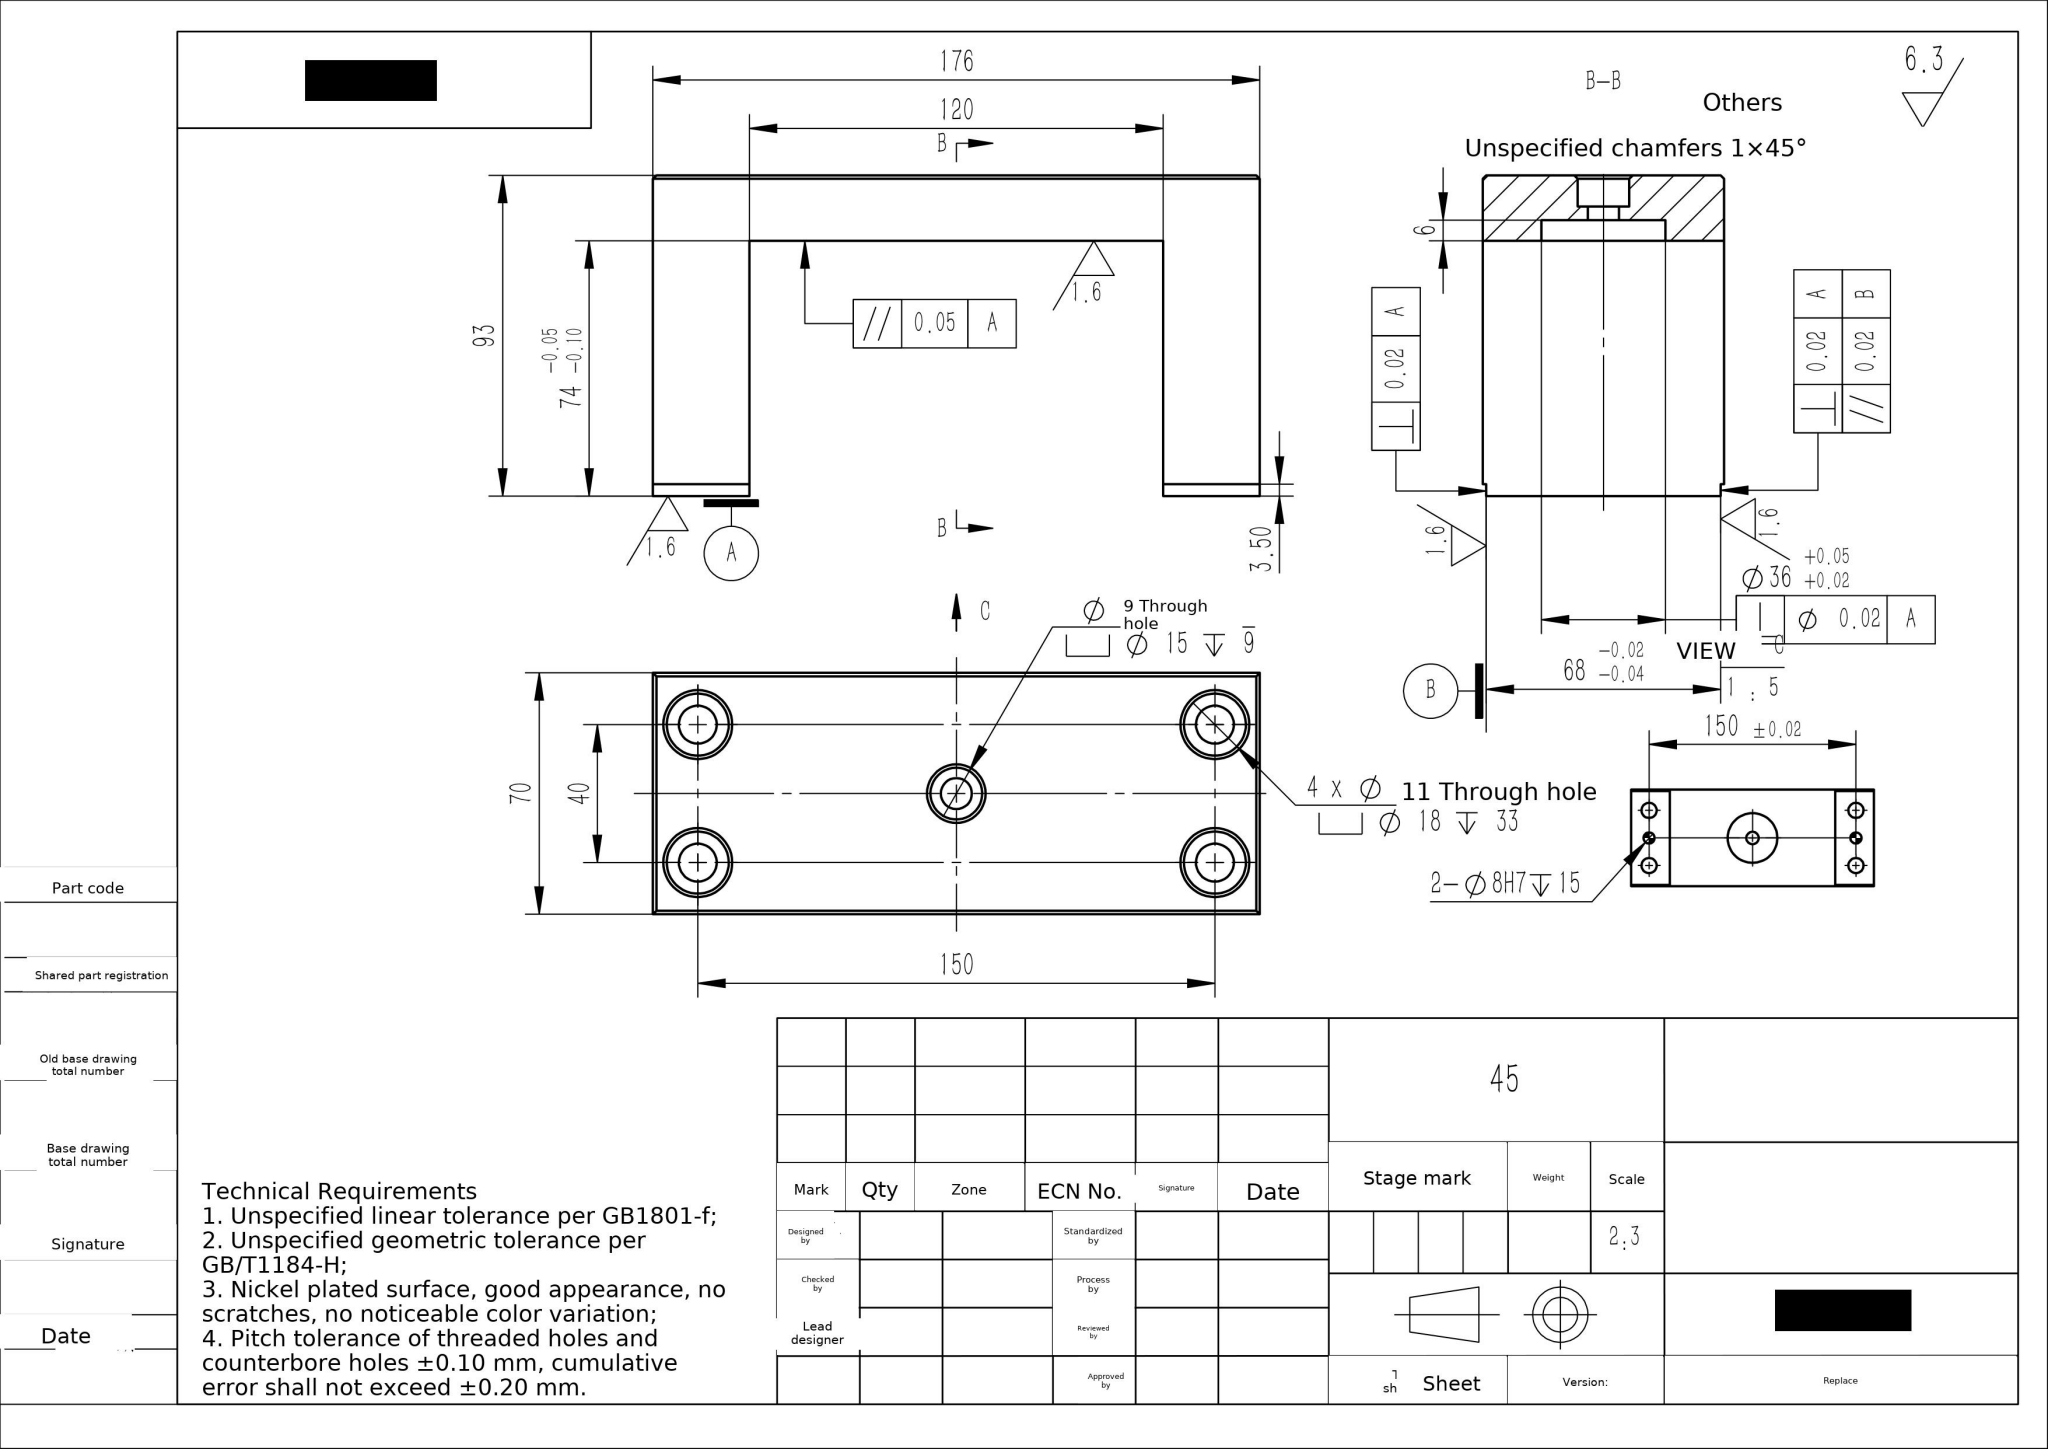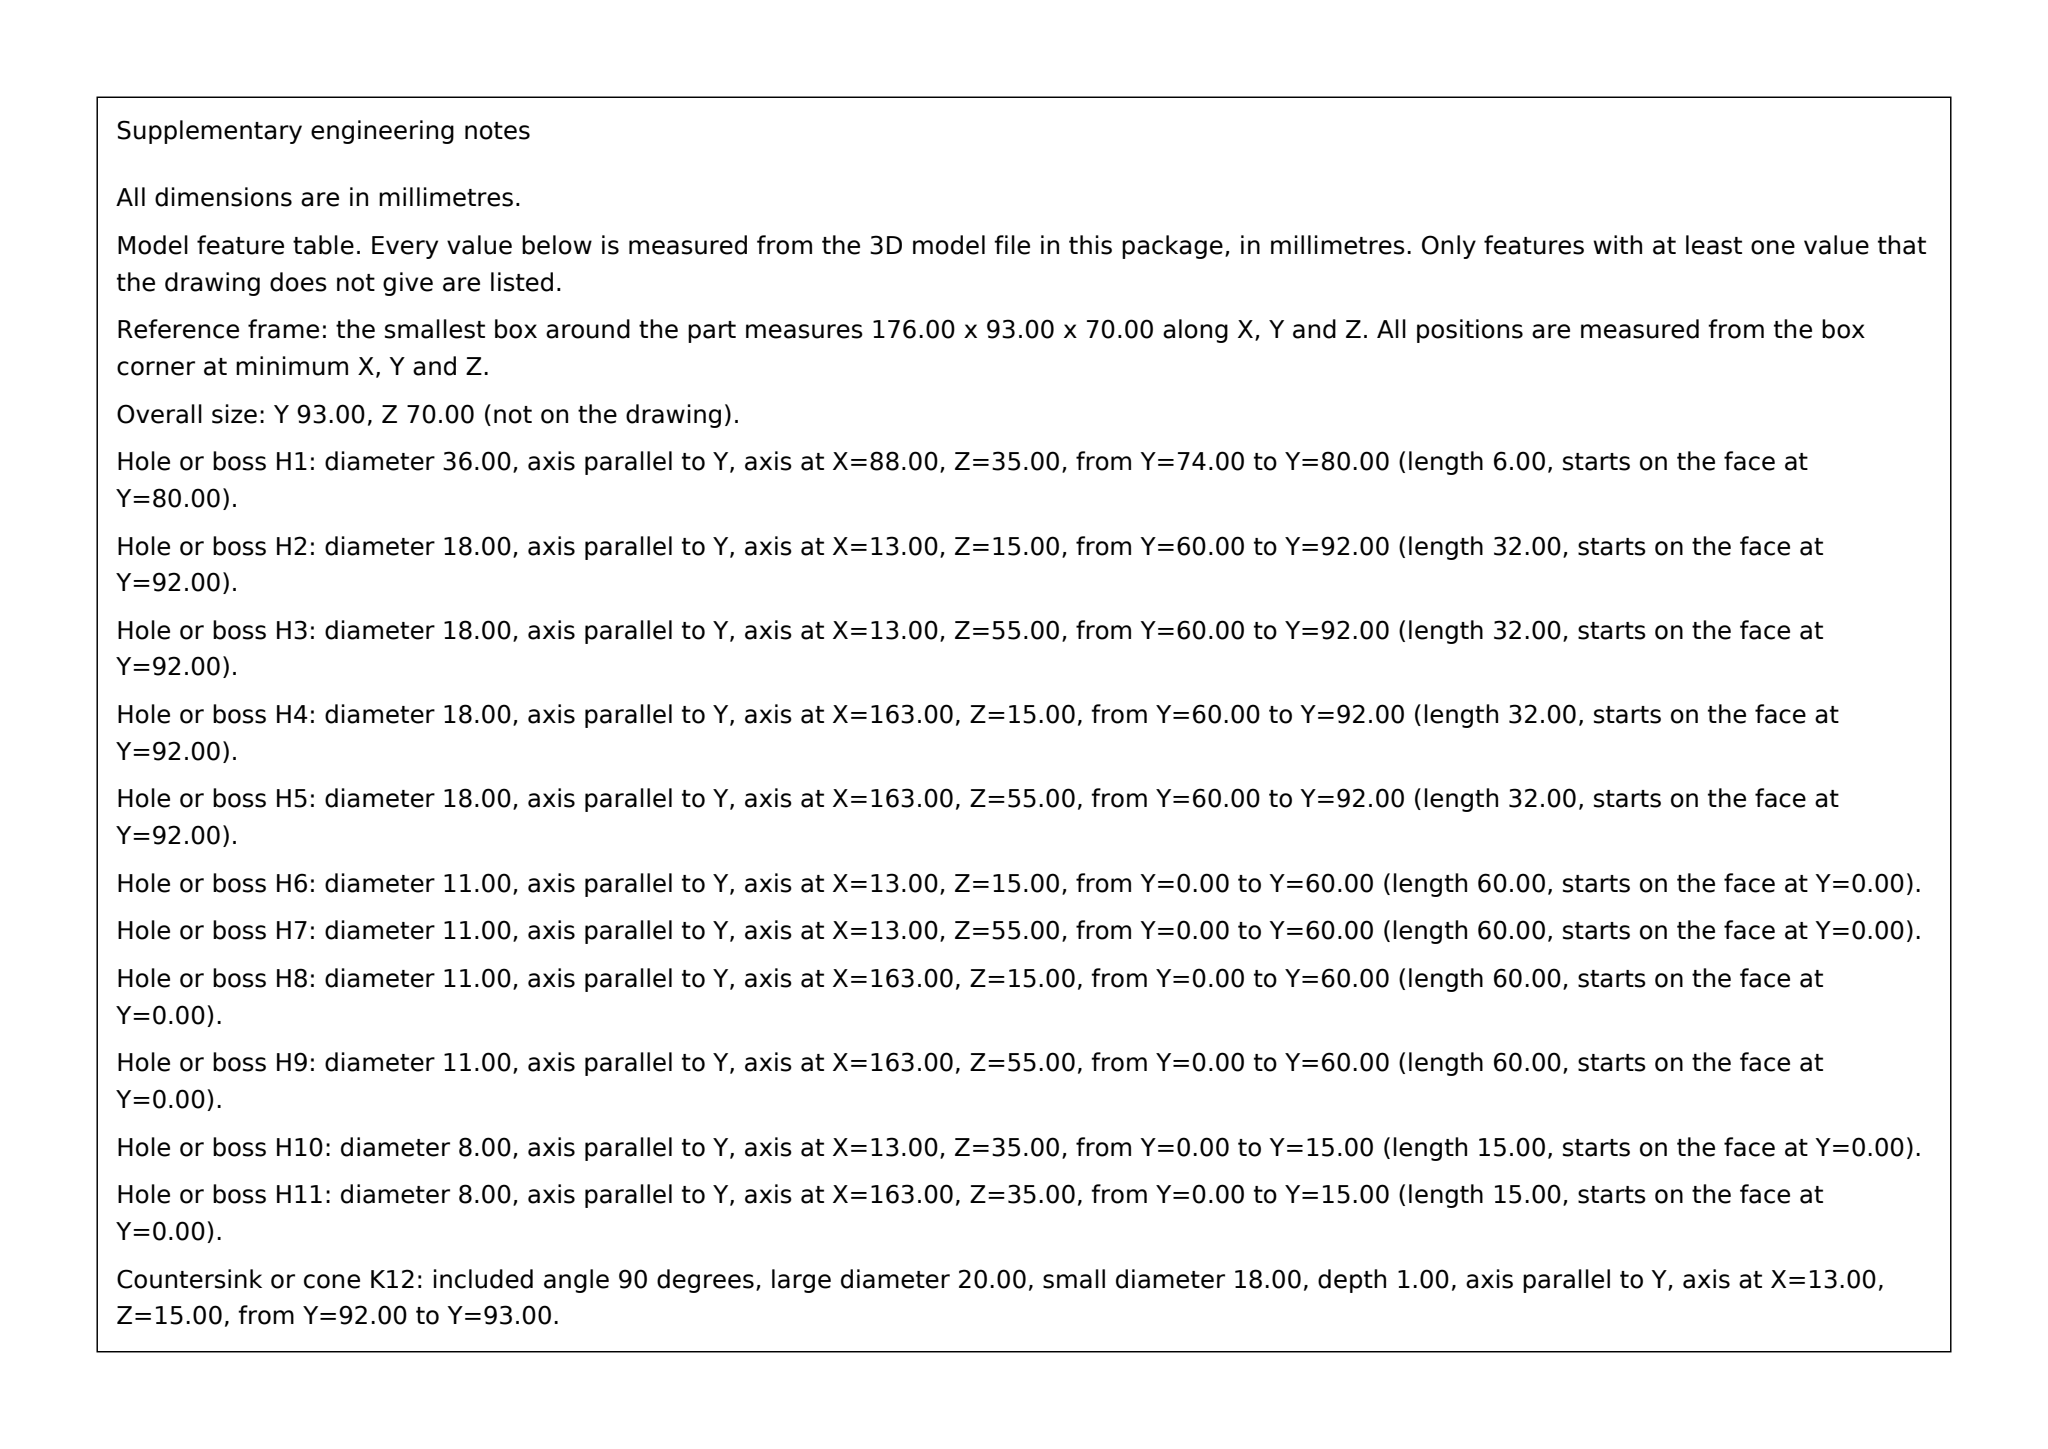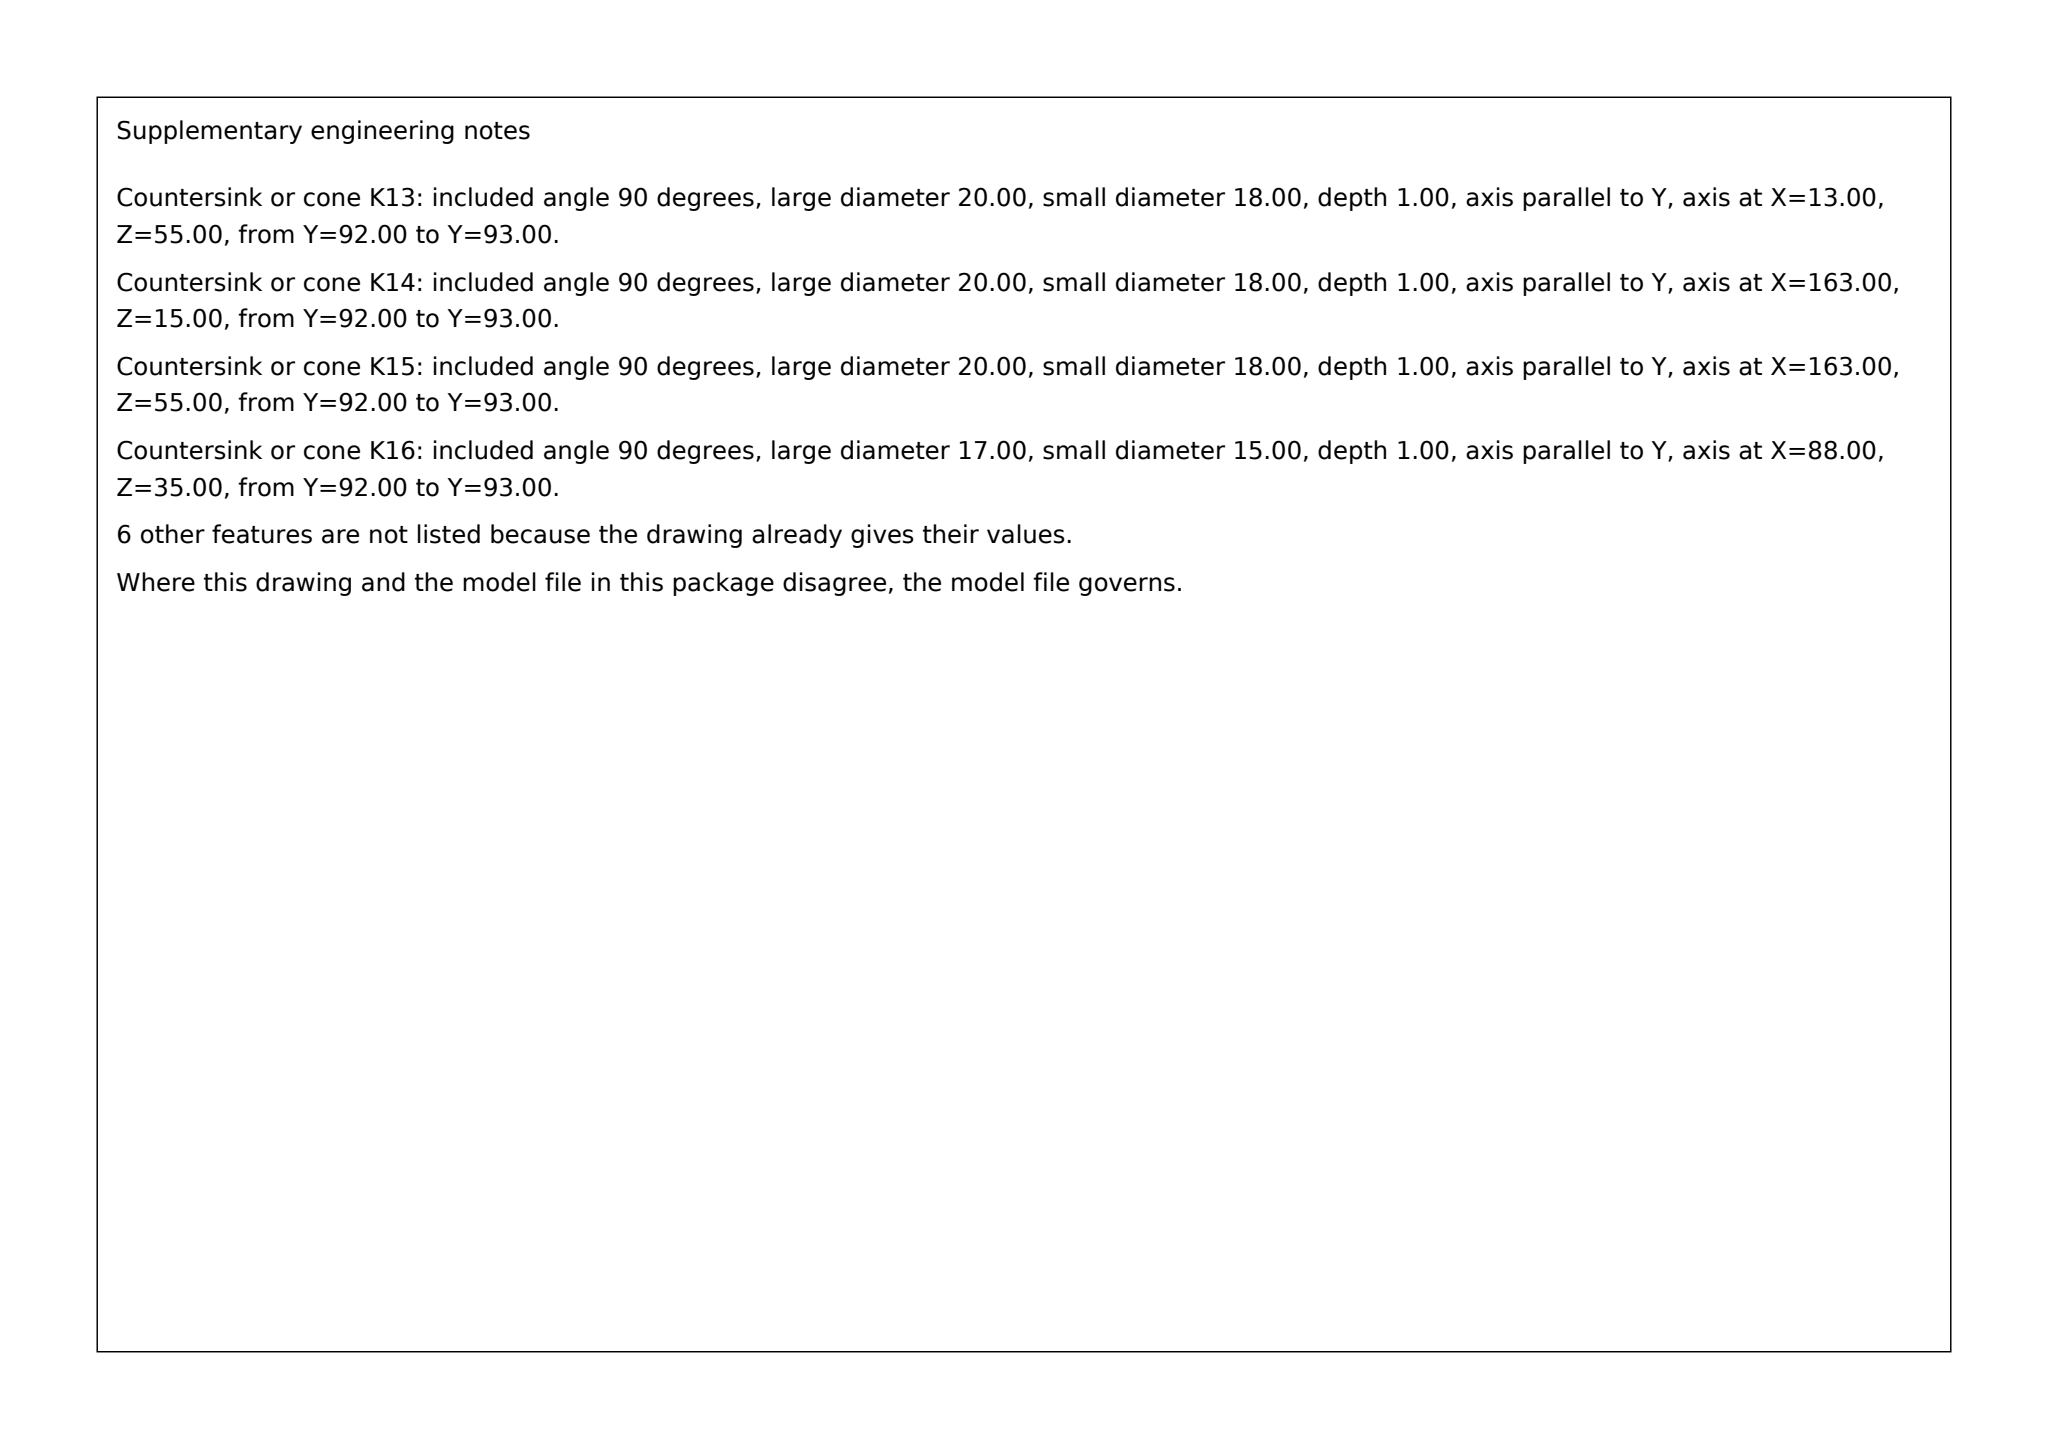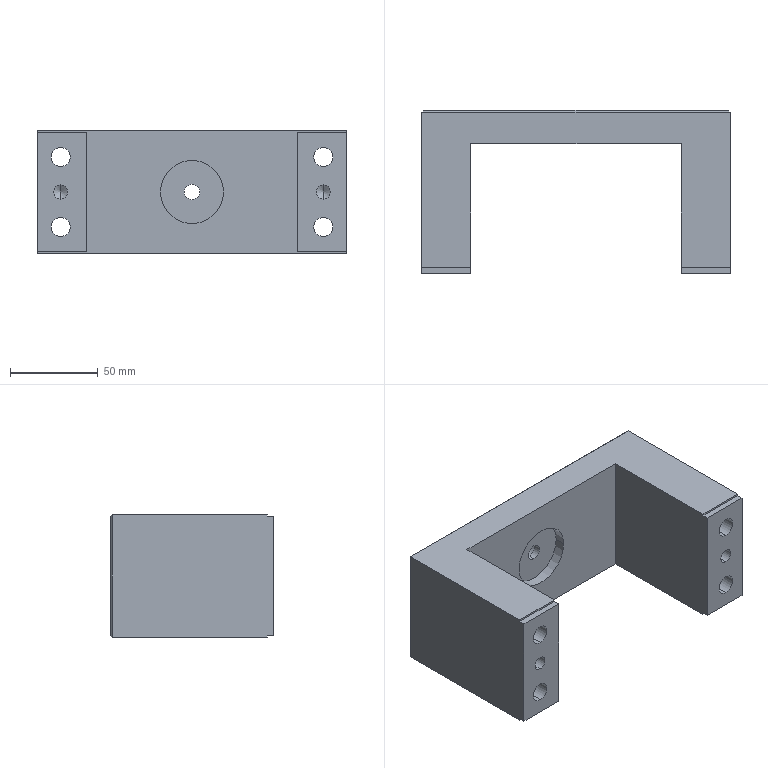Part | SolidWorks | mm | material 45 | 1 solid | 68 faces | box 176 x 93 x 70 mm | volume 457443 mm3 | plane 28 | cylinder 26 | cone 14 | commonest cylinder face diameters 18 x8 11 x8 8 x4 15 x2 9 x2 36 x2
build123d program:
from build123d import *

# Parameters (mm, degrees)
SKETCH1_W                                         = 176
SKETCH1_H                                         = 93
BOSS_EXTRUDE1_DEPTH                               = 70
SKETCH2_W                                         = 120
SKETCH2_H                                         = 148
CUT_EXTRUDE1_DEPTH                                = 122.681
SKETCH3_R                                         = 18
CUT_EXTRUDE2_DEPTH                                = 6
HOLE_SIZE_ACCORDING_TO_HEX_SOCKET_HEA_D           = 9
HOLE_SIZE_ACCORDING_TO_HEX_SOCKET_HEA_CBORE_D     = 15
HOLE_SIZE_ACCORDING_TO_HEX_SOCKET_HEA_CBORE_DEPTH = 9
HOLE_SIZE_ACCORDING_TO_HEX_SOCKET_2_D             = 11
HOLE_SIZE_ACCORDING_TO_HEX_SOCKET_2_CBORE_D       = 18
HOLE_SIZE_ACCORDING_TO_HEX_SOCKET_2_CBORE_DEPTH   = 33
CHAMFER1_SIZE                                     = 1
SKETCH16_W                                        = 176
SKETCH16_H                                        = 3.5
CUT_EXTRUDE3_DEPTH                                = 1


with BuildPart() as part:
    # Sketch1 → Boss-Extrude1 (new body)
    with BuildSketch(Plane.XY):
        Rectangle(SKETCH1_W, SKETCH1_H)
    extrude(amount=BOSS_EXTRUDE1_DEPTH)

    # Sketch2 → Cut-Extrude1 (cut, through all)
    with BuildSketch(Plane.XY.offset(70)):
        with Locations((0, -46.5)):
            Rectangle(SKETCH2_W, SKETCH2_H)
    extrude(amount=-CUT_EXTRUDE1_DEPTH, mode=Mode.SUBTRACT)

    # Sketch3 → Cut-Extrude2 (cut)
    with BuildSketch(Plane.XZ.offset(-27.5)):
        with Locations((0, 35)):
            Circle(SKETCH3_R)
    extrude(amount=-CUT_EXTRUDE2_DEPTH, mode=Mode.SUBTRACT)

    # Hole Size _ according to_ Hex Socket Hea (through all)
    with Locations(Plane(origin=(0, 46.5, 0), x_dir=(1, 0, 0), z_dir=(0, 1, 0))):
        with Locations((0, -35)):
            CounterBoreHole(HOLE_SIZE_ACCORDING_TO_HEX_SOCKET_HEA_D / 2, HOLE_SIZE_ACCORDING_TO_HEX_SOCKET_HEA_CBORE_D / 2, HOLE_SIZE_ACCORDING_TO_HEX_SOCKET_HEA_CBORE_DEPTH)

    # Hole Size _ according to_ Hex Socket 2 (through all)
    with Locations(Plane(origin=(0, 46.5, 0), x_dir=(1, 0, 0), z_dir=(0, 1, 0))):
        with Locations((-75, -15), (-75, -55)):
            hole_size_according_to_hex_socket_2 = CounterBoreHole(HOLE_SIZE_ACCORDING_TO_HEX_SOCKET_2_D / 2, HOLE_SIZE_ACCORDING_TO_HEX_SOCKET_2_CBORE_D / 2, HOLE_SIZE_ACCORDING_TO_HEX_SOCKET_2_CBORE_DEPTH)

    # Mirror1: Hole Size _ according to_ Hex Socket 2 across plane
    add(hole_size_according_to_hex_socket_2.mirror(Plane(origin=(0, 0, 0), x_dir=(0, 0, 1), z_dir=(1, 0, 0))), mode=Mode.SUBTRACT)

    # Chamfer1
    chamfer1_edges = [part.edges().sort_by_distance(p)[0] for p in [
        (-7.5, 46.5, 35),
        (-84, 46.5, 55),
        (0, 46.5, 0),
        (-84, 46.5, 15),
        (84, 46.5, 55),
        (84, 46.5, 15),
        (0, 46.5, 70),
        (-88, 46.5, 35),
        (88, 46.5, 35),
    ]]
    chamfer(chamfer1_edges, length=CHAMFER1_SIZE)

    # Sketch15 → Size mm Dowel Pin Hole1 (revolve, cut)
    with BuildSketch(Plane(origin=(-75, -46.5, 35), x_dir=(0, 0, -1), z_dir=(1, 0, 0))):
        Polygon((0, 0), (0, 17.403), (4, 15), (4, 0), align=None)
    size_mm_dowel_pin_hole1 = revolve(axis=Axis((-75, -52.85, 35), (0, 1, 0)), mode=Mode.SUBTRACT)

    # Mirror2: Size mm Dowel Pin Hole1 across plane
    add(size_mm_dowel_pin_hole1.mirror(Plane(origin=(0, 0, 0), x_dir=(0, 0, 1), z_dir=(1, 0, 0))), mode=Mode.SUBTRACT)

    # Sketch16 → Cut-Extrude3 (cut)
    with BuildSketch(Plane(origin=(0, 0, 0), x_dir=(-1, 0, 0), z_dir=(0, 0, -1))):
        with Locations((0, -44.75)):
            Rectangle(SKETCH16_W, SKETCH16_H)
    cut_extrude3 = extrude(amount=-CUT_EXTRUDE3_DEPTH, mode=Mode.SUBTRACT)

    # Mirror3: Cut-Extrude3 across plane
    add(cut_extrude3.mirror(Plane(origin=(0, 0, 35), x_dir=(1, 0, 0), z_dir=(0, 0, -1))), mode=Mode.SUBTRACT)


solid = part.part